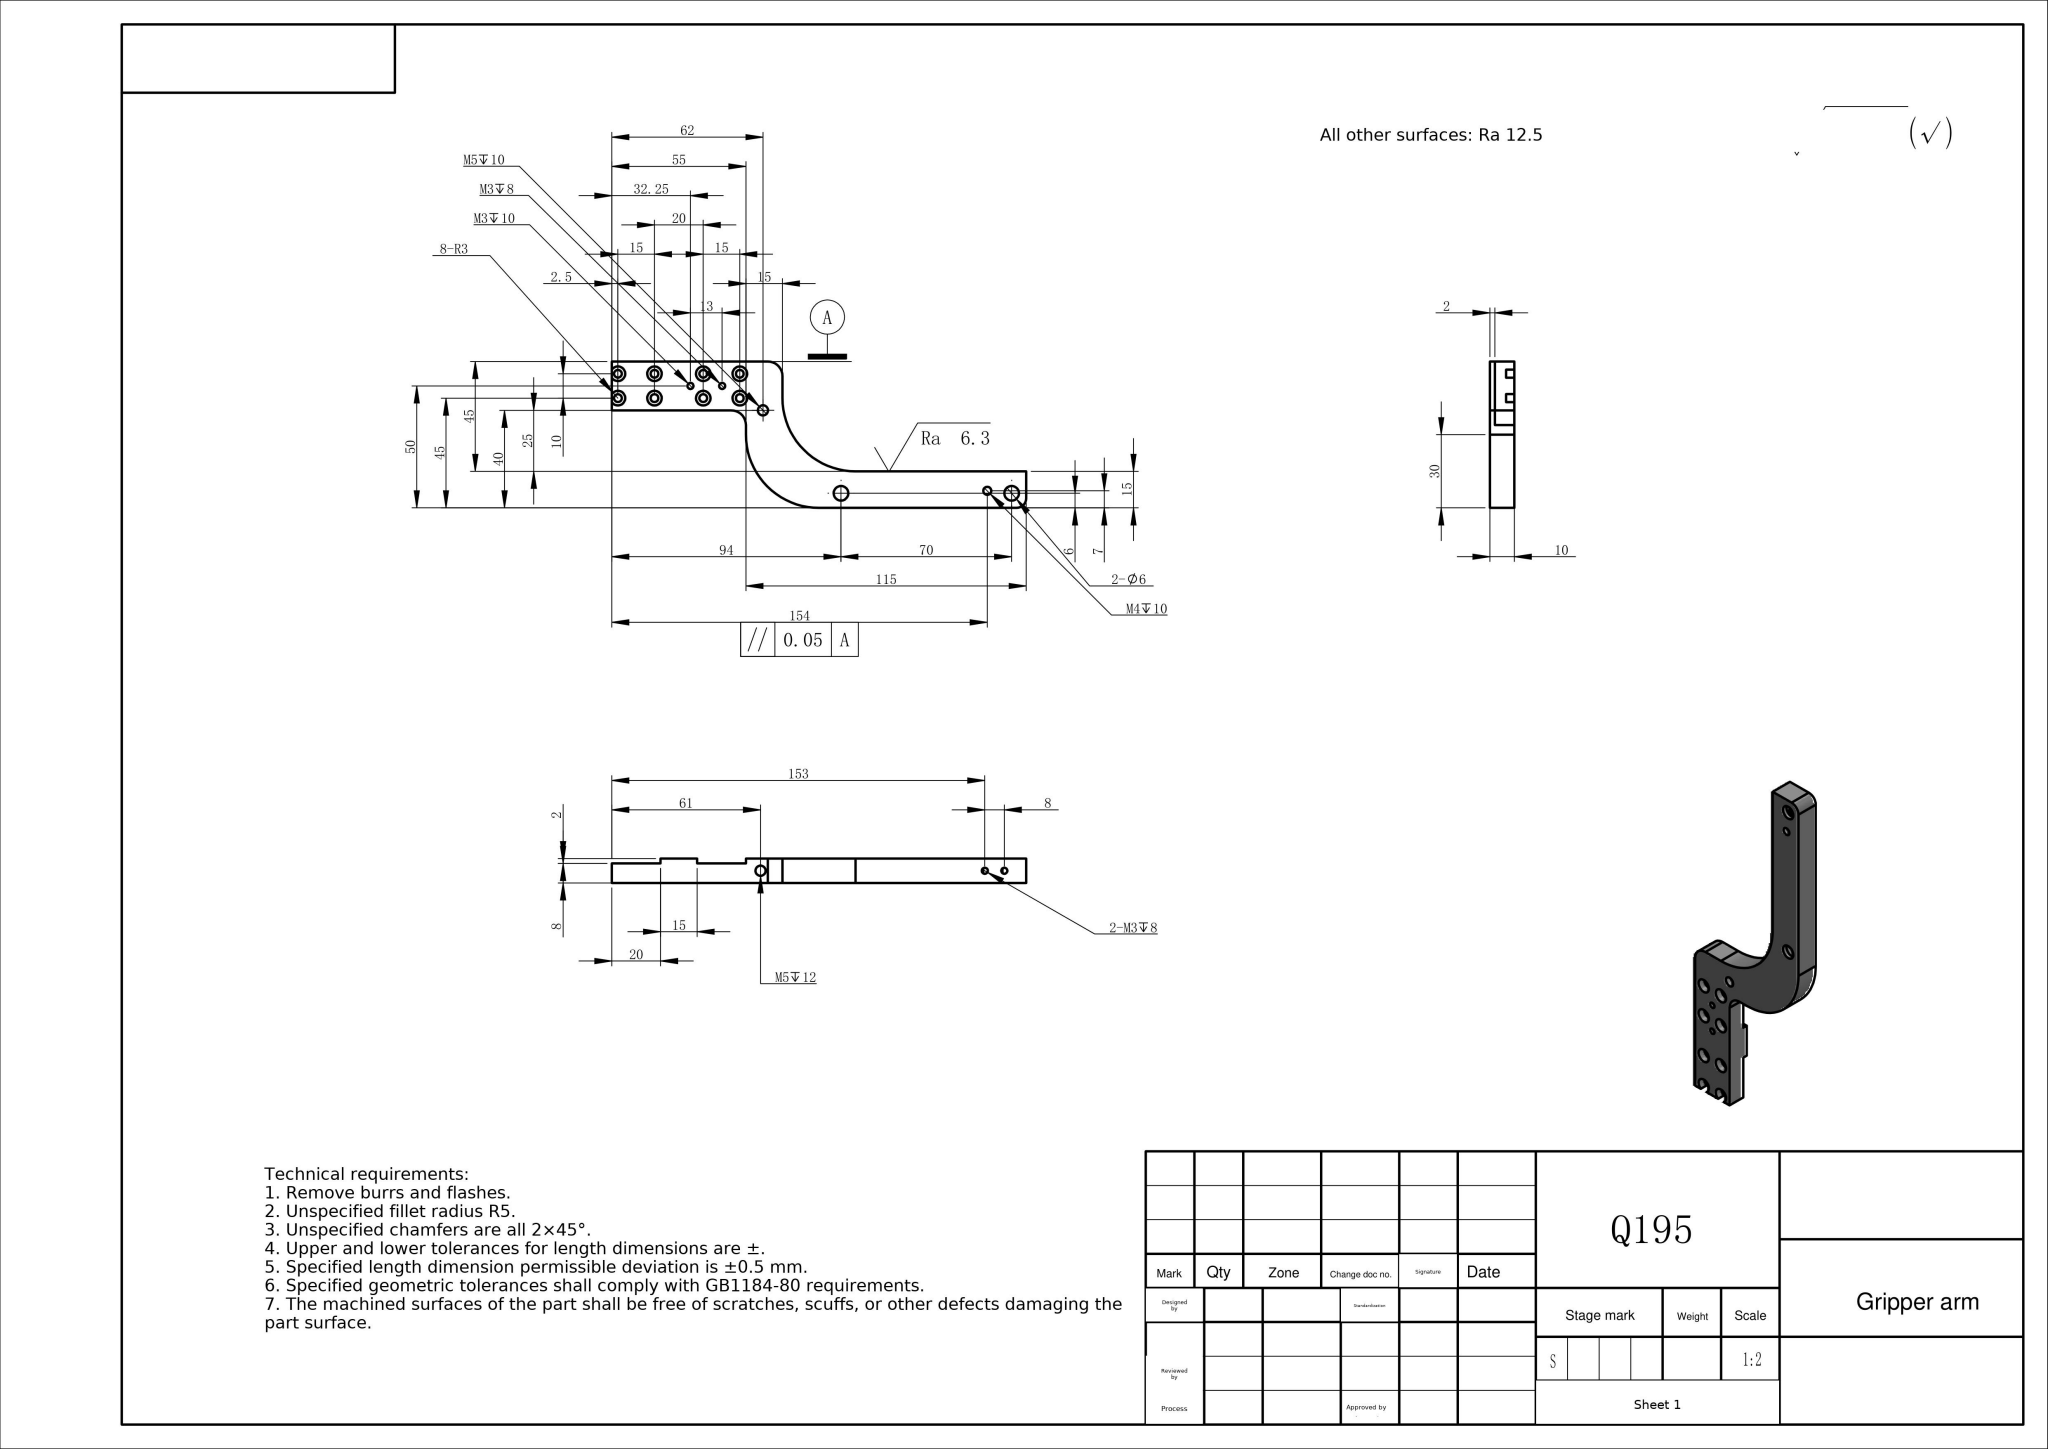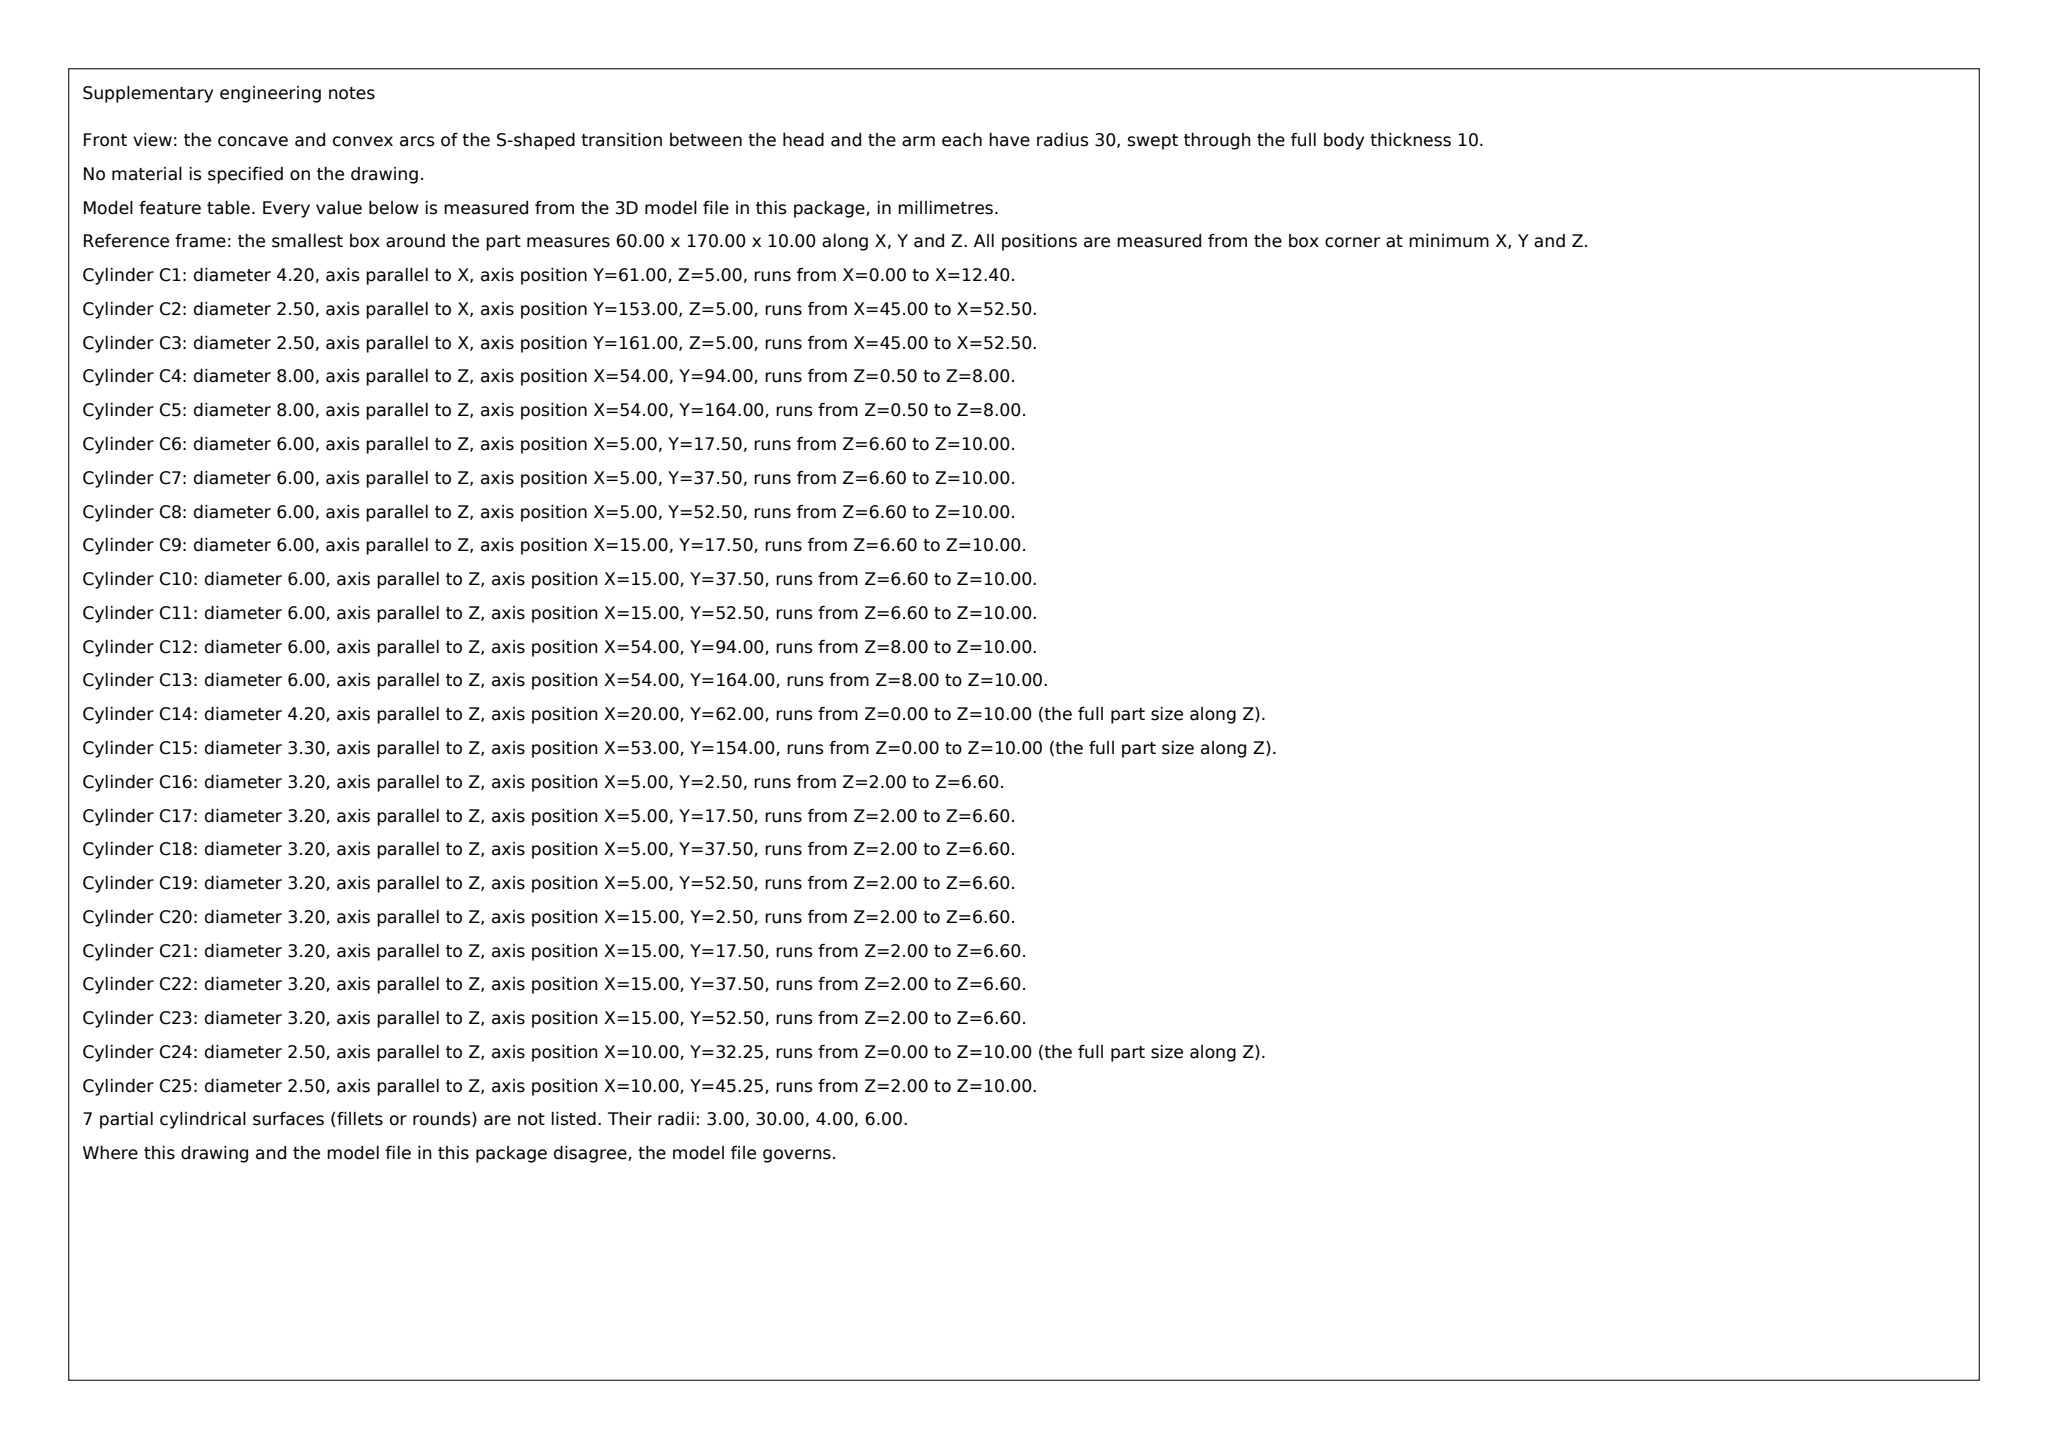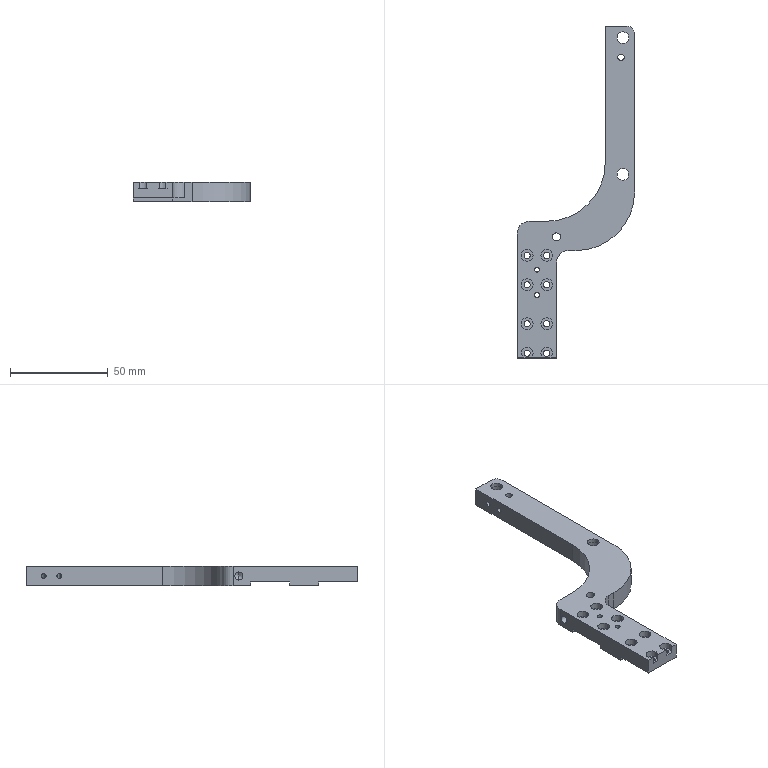Part | SolidWorks | mm | 1 solid | 94 faces | box 60 x 170 x 10 mm | volume 30817 mm3 | cylinder 61 | plane 25 | torus 4 | cone 4 | commonest cylinder face diameters 6 x22 3.2 x16 2.5 x8 8 x5 4.2 x4 3.3 x2 12 x2 60 x2
Drawing notes:
OVERALL LG 170; ARM END FACE 16 BEYOND M4 HOLE (154) | from the solid: bbox_xyz y=170; M4 tap drill O4.2 z-hole at y=62? no - M4 hole dia3.3 at y=154, end face plane y=170 -> 16
ARM TIP CNR R4, CTR 4 FROM END FACE & 4 FROM ARM OUTER EDGE | from the solid: cyl dia 8.0 axis z at [56,166] len 10 = full thk; tangent to x=60 and y=170 planes
2X R6: LEG OUTER CNR FULL 10 THK, STEP (20/55) INNER CNR R6 D8 | from the solid: cyl dia 12 axis z at [6,64] len 10 (tangent x=0,y=70); cyl dia 12 at [26,49] len 8 (tangent x=20,y=55)
M5 DP 12 & 2-M3 DP 8 AXES AT 5 FROM FACE, MID OF 10 THK | from the solid: x-axis cyls dia4.2 at [y=61,z=5] L12.4 and dia2.5 at [y=153,z=5],[y=161,z=5]; bbox z=10
LEG/BASE PLATE WIDTH 60 ACROSS HOLE-PATTERN FACE | from the solid: bbox_xyz x=60; planes x=0 and x=60 bound leg
8X Ø3.2 PATTERN: 2 ROWS AT 5 & 15 FROM PLATE EDGE (10 APART) | from the solid: Ø3.2 hole axes at x=5.0 and x=15.0; plane x=0 is face edge
M3 DP 8 AT 45.25 FROM END FACE (13 FROM M3 DP 10) | from the solid: Ø2.5 bore axis y=45.3, z 2.0-10.0 (depth 8); other at y=32.3 z 0-10
BACK STEP DP 2: 20 WIDE x 0-20 & 26 WIDE x 35-55 FROM END | from the solid: z=2 planes x[0,20] y[0,20] and x[0,26] y[35,55]; z=0 face x[0,20] y[20,35]
LEG END FACE 70 FROM BASE END; OUTER FACE 64 LG TO R6 TAN | from the solid: Plane y=70 (x 6-15, z 0-10); plane x=0 extent y 0-64; convex R6 arc ctr (6,64); concave R30 ctr (15,100)
4X R0.5 BLEND AT Ø8 C'BORE MOUTH | from the solid: tori minor_r 0.5, major_r 4.5, qty 4 at Ø8 bores (54,94) & (54,164)